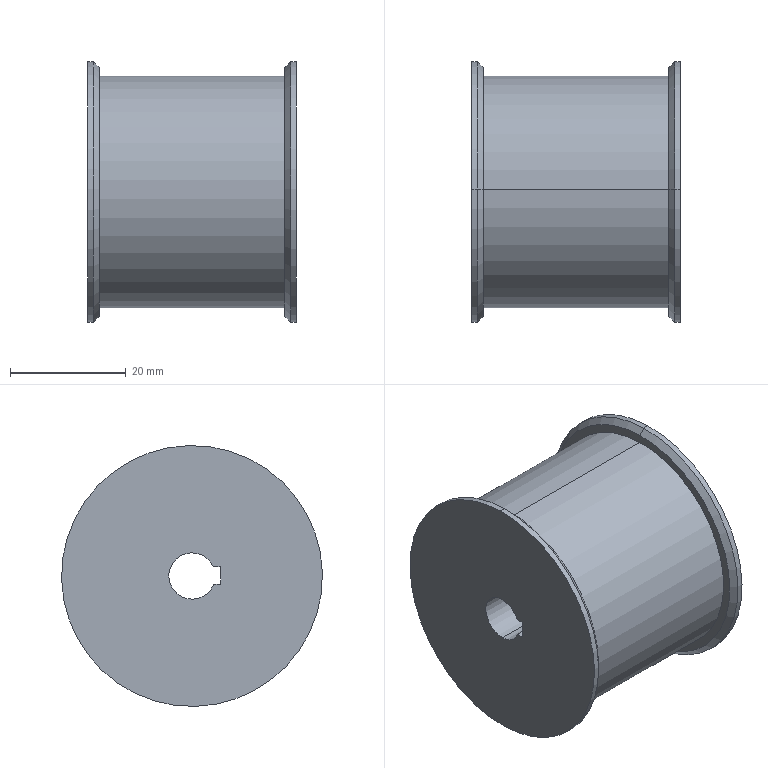Component | SolidWorks | CHEN123-AA-13-1 | 1 solid | 20 faces | box 36 x 45 x 45 mm | volume 44517 mm3 | cylinder 9 | plane 7 | cone 4 | commonest cylinder face diameters 45 x4 8 x3 40 x2
build123d program:
from build123d import *

# Parameters (mm, degrees)
SKETCH1_R           = 20
BOSS_EXTRUDE1_DEPTH = 16
SKETCH2_R           = 22.5
BOSS_EXTRUDE2_DEPTH = 2
BOSS_EXTRUDE3_START = 2
SKETCH3_R           = 22.5
BOSS_EXTRUDE3_DEPTH = 2
CHAMFER1_SIZE       = 1
SKETCH4_R           = 4
CUT_EXTRUDE1_DEPTH  = 49.047
SKETCH5_W           = 3
SKETCH5_H           = 1.816
CUT_EXTRUDE2_DEPTH  = 49.047


with BuildPart() as part:
    # Sketch1 → Boss-Extrude1 (new, symmetric)
    with BuildSketch(Plane.XY):
        Circle(SKETCH1_R)
    extrude(amount=BOSS_EXTRUDE1_DEPTH, both=True)

    # Sketch2 → Boss-Extrude2 (add)
    with BuildSketch(Plane.XY.offset(16)):
        Circle(SKETCH2_R)
    extrude(amount=BOSS_EXTRUDE2_DEPTH)

    # Sketch3 → Boss-Extrude3 (add)
    with BuildSketch(Plane(origin=(0, 0, -16), x_dir=(-1, 0, 0), z_dir=(0, 0, -1)).offset(BOSS_EXTRUDE3_START)):
        with Locations(Location((0, 0, 0), (0, 0, 180))):
            Circle(SKETCH3_R)
    extrude(amount=-BOSS_EXTRUDE3_DEPTH)

    # Chamfer1
    chamfer1_edges = [part.edges().sort_by_distance(p)[0] for p in [
        (-22.5, 0, 16),
        (-22.5, 0, -16),
    ]]
    chamfer(chamfer1_edges, length=CHAMFER1_SIZE)

    # Sketch4 → Cut-Extrude1 (cut, through all)
    with BuildSketch(Plane(origin=(0, 0, -18), x_dir=(-1, 0, 0), z_dir=(0, 0, -1))):
        Circle(SKETCH4_R)
    extrude(amount=-CUT_EXTRUDE1_DEPTH, mode=Mode.SUBTRACT)

    # Sketch5 → Cut-Extrude2 (cut, through all)
    with BuildSketch(Plane(origin=(0, 0, -18), x_dir=(-1, 0, 0), z_dir=(0, 0, -1))):
        with Locations((0, 4)):
            Rectangle(SKETCH5_W, SKETCH5_H)
    extrude(amount=-CUT_EXTRUDE2_DEPTH, mode=Mode.SUBTRACT)


solid = part.part

# Placed as in the assembly
solid = solid.moved(Location((-0.0005, -95.999, -200), (178.787, -90, 0)))
STEP:
#1=CARTESIAN_POINT('',(-0.7087,-3.783,-8.031));
#2=VERTEX_POINT('',#1);
#3=CARTESIAN_POINT('',(-0.7087,-3.776,-7.717));
#4=VERTEX_POINT('',#3);
#5=CARTESIAN_POINT('',(-0.7087,-3.779,-7.874));
#6=DIRECTION('',(1.,0.,0.));
#7=DIRECTION('',(0.,0.02117,0.9998));
#8=AXIS2_PLACEMENT_3D('',#5,#6,#7);
#9=CIRCLE('',#8,0.1575);
#10=EDGE_CURVE('',#2,#4,#9,.T.);
#11=ORIENTED_EDGE('',*,*,#10,.F.);
#12=CARTESIAN_POINT('',(0.7086,-3.783,-8.031));
#13=VERTEX_POINT('',#12);
#14=CARTESIAN_POINT('',(-0.7087,-3.783,-8.031));
#15=DIRECTION('',(1.,0.,0.));
#16=VECTOR('',#15,39.37);
#17=LINE('',#14,#16);
#18=EDGE_CURVE('',#2,#13,#17,.T.);
#19=ORIENTED_EDGE('',*,*,#18,.T.);
#20=CARTESIAN_POINT('',(0.7086,-3.776,-7.717));
#21=VERTEX_POINT('',#20);
#22=CARTESIAN_POINT('',(0.7086,-3.779,-7.874));
#23=DIRECTION('',(1.,0.,0.));
#24=DIRECTION('',(0.,0.02117,0.9998));
#25=AXIS2_PLACEMENT_3D('',#22,#23,#24);
#26=CIRCLE('',#25,0.1575);
#27=EDGE_CURVE('',#13,#21,#26,.T.);
#28=ORIENTED_EDGE('',*,*,#27,.T.);
#29=CARTESIAN_POINT('',(-0.7087,-3.776,-7.717));
#30=DIRECTION('',(1.,0.,0.));
#31=VECTOR('',#30,39.37);
#32=LINE('',#29,#31);
#33=EDGE_CURVE('',#4,#21,#32,.T.);
#34=ORIENTED_EDGE('',*,*,#33,.F.);
#35=EDGE_LOOP('',(#11,#19,#28,#34));
#36=FACE_OUTER_BOUND('',#35,.T.);
#37=CARTESIAN_POINT('',(-0.7087,-3.779,-7.874));
#38=DIRECTION('',(1.,0.,0.));
#39=DIRECTION('',(0.,0.02117,0.9998));
#40=AXIS2_PLACEMENT_3D('',#37,#38,#39);
#41=CYLINDRICAL_SURFACE('',#40,0.1575);
#42=ADVANCED_FACE('',(#36),#41,.F.);
#43=CARTESIAN_POINT('',(-0.7087,-3.924,-7.812));
#44=VERTEX_POINT('',#43);
#45=CARTESIAN_POINT('',(-0.7087,-3.779,-7.874));
#46=DIRECTION('',(1.,0.,0.));
#47=DIRECTION('',(0.,0.02117,0.9998));
#48=AXIS2_PLACEMENT_3D('',#45,#46,#47);
#49=CIRCLE('',#48,0.1575);
#50=EDGE_CURVE('',#4,#44,#49,.T.);
#51=ORIENTED_EDGE('',*,*,#50,.F.);
#52=ORIENTED_EDGE('',*,*,#33,.T.);
#53=CARTESIAN_POINT('',(0.7086,-3.924,-7.812));
#54=VERTEX_POINT('',#53);
#55=CARTESIAN_POINT('',(0.7086,-3.779,-7.874));
#56=DIRECTION('',(1.,0.,0.));
#57=DIRECTION('',(0.,0.02117,0.9998));
#58=AXIS2_PLACEMENT_3D('',#55,#56,#57);
#59=CIRCLE('',#58,0.1575);
#60=EDGE_CURVE('',#21,#54,#59,.T.);
#61=ORIENTED_EDGE('',*,*,#60,.T.);
#62=CARTESIAN_POINT('',(-0.7087,-3.924,-7.812));
#63=DIRECTION('',(-1.,0.,0.));
#64=VECTOR('',#63,39.37);
#65=LINE('',#62,#64);
#66=EDGE_CURVE('',#54,#44,#65,.T.);
#67=ORIENTED_EDGE('',*,*,#66,.T.);
#68=EDGE_LOOP('',(#51,#52,#61,#67));
#69=FACE_OUTER_BOUND('',#68,.T.);
#70=CARTESIAN_POINT('',(-0.7087,-3.779,-7.874));
#71=DIRECTION('',(1.,0.,0.));
#72=DIRECTION('',(0.,0.02117,0.9998));
#73=AXIS2_PLACEMENT_3D('',#70,#71,#72);
#74=CYLINDRICAL_SURFACE('',#73,0.1575);
#75=ADVANCED_FACE('',(#69),#74,.F.);
#76=CARTESIAN_POINT('',(-0.6299,-3.762,-7.028));
#77=VERTEX_POINT('',#76);
#78=CARTESIAN_POINT('',(-0.6299,-3.797,-8.72));
#79=VERTEX_POINT('',#78);
#80=CARTESIAN_POINT('',(-0.6299,-3.779,-7.874));
#81=DIRECTION('',(1.,0.,0.));
#82=DIRECTION('',(0.,-0.02117,-0.9998));
#83=AXIS2_PLACEMENT_3D('',#80,#81,#82);
#84=CIRCLE('',#83,0.8465);
#85=EDGE_CURVE('',#77,#79,#84,.T.);
#86=ORIENTED_EDGE('',*,*,#85,.F.);
#87=CARTESIAN_POINT('',(-0.6693,-3.761,-6.988));
#88=VERTEX_POINT('',#87);
#89=CARTESIAN_POINT('',(-0.6693,-3.761,-6.988));
#90=DIRECTION('',(-0.7071,0.01497,0.7069));
#91=VECTOR('',#90,39.37);
#92=LINE('',#89,#91);
#93=EDGE_CURVE('',#77,#88,#92,.T.);
#94=ORIENTED_EDGE('',*,*,#93,.T.);
#95=CARTESIAN_POINT('',(-0.6693,-3.798,-8.76));
#96=VERTEX_POINT('',#95);
#97=CARTESIAN_POINT('',(-0.6693,-3.779,-7.874));
#98=DIRECTION('',(-1.,0.,0.));
#99=DIRECTION('',(0.,-0.02117,-0.9998));
#100=AXIS2_PLACEMENT_3D('',#97,#98,#99);
#101=CIRCLE('',#100,0.8858);
#102=EDGE_CURVE('',#96,#88,#101,.T.);
#103=ORIENTED_EDGE('',*,*,#102,.F.);
#104=CARTESIAN_POINT('',(-0.6693,-3.798,-8.76));
#105=DIRECTION('',(-0.7071,-0.01497,-0.7069));
#106=VECTOR('',#105,39.37);
#107=LINE('',#104,#106);
#108=EDGE_CURVE('',#79,#96,#107,.T.);
#109=ORIENTED_EDGE('',*,*,#108,.F.);
#110=EDGE_LOOP('',(#86,#94,#103,#109));
#111=FACE_OUTER_BOUND('',#110,.T.);
#112=CARTESIAN_POINT('',(-0.6693,-3.779,-7.874));
#113=DIRECTION('',(-1.,0.,0.));
#114=DIRECTION('',(0.,-0.02117,-0.9998));
#115=AXIS2_PLACEMENT_3D('',#112,#113,#114);
#116=CONICAL_SURFACE('',#115,0.8858,0.7854);
#117=ADVANCED_FACE('',(#111),#116,.T.);
#118=CARTESIAN_POINT('',(0.6299,-3.797,-8.72));
#119=VERTEX_POINT('',#118);
#120=CARTESIAN_POINT('',(0.6299,-3.762,-7.028));
#121=VERTEX_POINT('',#120);
#122=CARTESIAN_POINT('',(0.6299,-3.779,-7.874));
#123=DIRECTION('',(-1.,0.,0.));
#124=DIRECTION('',(0.,0.02117,0.9998));
#125=AXIS2_PLACEMENT_3D('',#122,#123,#124);
#126=CIRCLE('',#125,0.8465);
#127=EDGE_CURVE('',#119,#121,#126,.T.);
#128=ORIENTED_EDGE('',*,*,#127,.F.);
#129=CARTESIAN_POINT('',(0.6693,-3.798,-8.76));
#130=VERTEX_POINT('',#129);
#131=CARTESIAN_POINT('',(0.6693,-3.798,-8.76));
#132=DIRECTION('',(0.7071,-0.01497,-0.7069));
#133=VECTOR('',#132,39.37);
#134=LINE('',#131,#133);
#135=EDGE_CURVE('',#119,#130,#134,.T.);
#136=ORIENTED_EDGE('',*,*,#135,.T.);
#137=CARTESIAN_POINT('',(0.6693,-3.761,-6.988));
#138=VERTEX_POINT('',#137);
#139=CARTESIAN_POINT('',(0.6693,-3.779,-7.874));
#140=DIRECTION('',(1.,0.,0.));
#141=DIRECTION('',(0.,0.02117,0.9998));
#142=AXIS2_PLACEMENT_3D('',#139,#140,#141);
#143=CIRCLE('',#142,0.8858);
#144=EDGE_CURVE('',#138,#130,#143,.T.);
#145=ORIENTED_EDGE('',*,*,#144,.F.);
#146=CARTESIAN_POINT('',(0.6693,-3.761,-6.988));
#147=DIRECTION('',(0.7071,0.01497,0.7069));
#148=VECTOR('',#147,39.37);
#149=LINE('',#146,#148);
#150=EDGE_CURVE('',#121,#138,#149,.T.);
#151=ORIENTED_EDGE('',*,*,#150,.F.);
#152=EDGE_LOOP('',(#128,#136,#145,#151));
#153=FACE_OUTER_BOUND('',#152,.T.);
#154=CARTESIAN_POINT('',(0.6693,-3.779,-7.874));
#155=DIRECTION('',(1.,0.,0.));
#156=DIRECTION('',(0.,0.02117,0.9998));
#157=AXIS2_PLACEMENT_3D('',#154,#155,#156);
#158=CONICAL_SURFACE('',#157,0.8858,0.7854);
#159=ADVANCED_FACE('',(#153),#158,.T.);
#160=CARTESIAN_POINT('',(0.7086,-3.761,-6.988));
#161=VERTEX_POINT('',#160);
#162=CARTESIAN_POINT('',(0.7086,-3.798,-8.76));
#163=VERTEX_POINT('',#162);
#164=CARTESIAN_POINT('',(0.7086,-3.779,-7.874));
#165=DIRECTION('',(1.,0.,0.));
#166=DIRECTION('',(0.,0.02117,0.9998));
#167=AXIS2_PLACEMENT_3D('',#164,#165,#166);
#168=CIRCLE('',#167,0.8858);
#169=EDGE_CURVE('',#161,#163,#168,.T.);
#170=ORIENTED_EDGE('',*,*,#169,.F.);
#171=CARTESIAN_POINT('',(0.7086,-3.761,-6.988));
#172=DIRECTION('',(-1.,0.,0.));
#173=VECTOR('',#172,39.37);
#174=LINE('',#171,#173);
#175=EDGE_CURVE('',#161,#138,#174,.T.);
#176=ORIENTED_EDGE('',*,*,#175,.T.);
#177=ORIENTED_EDGE('',*,*,#144,.T.);
#178=CARTESIAN_POINT('',(0.7086,-3.798,-8.76));
#179=DIRECTION('',(-1.,0.,0.));
#180=VECTOR('',#179,39.37);
#181=LINE('',#178,#180);
#182=EDGE_CURVE('',#163,#130,#181,.T.);
#183=ORIENTED_EDGE('',*,*,#182,.F.);
#184=EDGE_LOOP('',(#170,#176,#177,#183));
#185=FACE_OUTER_BOUND('',#184,.T.);
#186=CARTESIAN_POINT('',(0.7086,-3.779,-7.874));
#187=DIRECTION('',(-1.,0.,0.));
#188=DIRECTION('',(0.,-0.02117,-0.9998));
#189=AXIS2_PLACEMENT_3D('',#186,#187,#188);
#190=CYLINDRICAL_SURFACE('',#189,0.8858);
#191=ADVANCED_FACE('',(#185),#190,.T.);
#192=CARTESIAN_POINT('',(-0.7087,-3.798,-8.76));
#193=VERTEX_POINT('',#192);
#194=CARTESIAN_POINT('',(-0.7087,-3.761,-6.988));
#195=VERTEX_POINT('',#194);
#196=CARTESIAN_POINT('',(-0.7087,-3.779,-7.874));
#197=DIRECTION('',(-1.,0.,0.));
#198=DIRECTION('',(0.,-0.02117,-0.9998));
#199=AXIS2_PLACEMENT_3D('',#196,#197,#198);
#200=CIRCLE('',#199,0.8858);
#201=EDGE_CURVE('',#193,#195,#200,.T.);
#202=ORIENTED_EDGE('',*,*,#201,.F.);
#203=CARTESIAN_POINT('',(-0.7087,-3.798,-8.76));
#204=DIRECTION('',(1.,0.,0.));
#205=VECTOR('',#204,39.37);
#206=LINE('',#203,#205);
#207=EDGE_CURVE('',#193,#96,#206,.T.);
#208=ORIENTED_EDGE('',*,*,#207,.T.);
#209=ORIENTED_EDGE('',*,*,#102,.T.);
#210=CARTESIAN_POINT('',(-0.7087,-3.761,-6.988));
#211=DIRECTION('',(1.,0.,0.));
#212=VECTOR('',#211,39.37);
#213=LINE('',#210,#212);
#214=EDGE_CURVE('',#195,#88,#213,.T.);
#215=ORIENTED_EDGE('',*,*,#214,.F.);
#216=EDGE_LOOP('',(#202,#208,#209,#215));
#217=FACE_OUTER_BOUND('',#216,.T.);
#218=CARTESIAN_POINT('',(-0.7087,-3.779,-7.874));
#219=DIRECTION('',(1.,0.,0.));
#220=DIRECTION('',(0.,0.02117,0.9998));
#221=AXIS2_PLACEMENT_3D('',#218,#219,#220);
#222=CYLINDRICAL_SURFACE('',#221,0.8858);
#223=ADVANCED_FACE('',(#217),#222,.T.);
#224=CARTESIAN_POINT('',(-0.6299,-3.796,-8.661));
#225=VERTEX_POINT('',#224);
#226=CARTESIAN_POINT('',(-0.6299,-3.763,-7.087));
#227=VERTEX_POINT('',#226);
#228=CARTESIAN_POINT('',(-0.6299,-3.779,-7.874));
#229=DIRECTION('',(-1.,0.,0.));
#230=DIRECTION('',(0.,-0.02117,-0.9998));
#231=AXIS2_PLACEMENT_3D('',#228,#229,#230);
#232=CIRCLE('',#231,0.7874);
#233=EDGE_CURVE('',#225,#227,#232,.T.);
#234=ORIENTED_EDGE('',*,*,#233,.F.);
#235=CARTESIAN_POINT('',(0.6299,-3.796,-8.661));
#236=VERTEX_POINT('',#235);
#237=CARTESIAN_POINT('',(-0.6299,-3.796,-8.661));
#238=DIRECTION('',(1.,0.,0.));
#239=VECTOR('',#238,39.37);
#240=LINE('',#237,#239);
#241=EDGE_CURVE('',#225,#236,#240,.T.);
#242=ORIENTED_EDGE('',*,*,#241,.T.);
#243=CARTESIAN_POINT('',(0.6299,-3.763,-7.087));
#244=VERTEX_POINT('',#243);
#245=CARTESIAN_POINT('',(0.6299,-3.779,-7.874));
#246=DIRECTION('',(-1.,0.,0.));
#247=DIRECTION('',(0.,-0.02117,-0.9998));
#248=AXIS2_PLACEMENT_3D('',#245,#246,#247);
#249=CIRCLE('',#248,0.7874);
#250=EDGE_CURVE('',#236,#244,#249,.T.);
#251=ORIENTED_EDGE('',*,*,#250,.T.);
#252=CARTESIAN_POINT('',(-0.6299,-3.763,-7.087));
#253=DIRECTION('',(1.,0.,0.));
#254=VECTOR('',#253,39.37);
#255=LINE('',#252,#254);
#256=EDGE_CURVE('',#227,#244,#255,.T.);
#257=ORIENTED_EDGE('',*,*,#256,.F.);
#258=EDGE_LOOP('',(#234,#242,#251,#257));
#259=FACE_OUTER_BOUND('',#258,.T.);
#260=CARTESIAN_POINT('',(-0.6299,-3.779,-7.874));
#261=DIRECTION('',(1.,0.,0.));
#262=DIRECTION('',(0.,0.02117,0.9998));
#263=AXIS2_PLACEMENT_3D('',#260,#261,#262);
#264=CYLINDRICAL_SURFACE('',#263,0.7874);
#265=ADVANCED_FACE('',(#259),#264,.T.);
#266=ORIENTED_EDGE('',*,*,#241,.F.);
#267=CARTESIAN_POINT('',(-0.6299,-3.779,-7.874));
#268=DIRECTION('',(-1.,0.,0.));
#269=DIRECTION('',(0.,-0.02117,-0.9998));
#270=AXIS2_PLACEMENT_3D('',#267,#268,#269);
#271=CIRCLE('',#270,0.7874);
#272=EDGE_CURVE('',#227,#225,#271,.T.);
#273=ORIENTED_EDGE('',*,*,#272,.F.);
#274=ORIENTED_EDGE('',*,*,#256,.T.);
#275=CARTESIAN_POINT('',(0.6299,-3.779,-7.874));
#276=DIRECTION('',(-1.,0.,0.));
#277=DIRECTION('',(0.,-0.02117,-0.9998));
#278=AXIS2_PLACEMENT_3D('',#275,#276,#277);
#279=CIRCLE('',#278,0.7874);
#280=EDGE_CURVE('',#244,#236,#279,.T.);
#281=ORIENTED_EDGE('',*,*,#280,.T.);
#282=EDGE_LOOP('',(#266,#273,#274,#281));
#283=FACE_OUTER_BOUND('',#282,.T.);
#284=CARTESIAN_POINT('',(-0.6299,-3.779,-7.874));
#285=DIRECTION('',(1.,0.,0.));
#286=DIRECTION('',(0.,0.02117,0.9998));
#287=AXIS2_PLACEMENT_3D('',#284,#285,#286);
#288=CYLINDRICAL_SURFACE('',#287,0.7874);
#289=ADVANCED_FACE('',(#283),#288,.T.);
#290=ORIENTED_EDGE('',*,*,#207,.F.);
#291=CARTESIAN_POINT('',(-0.7087,-3.779,-7.874));
#292=DIRECTION('',(-1.,0.,0.));
#293=DIRECTION('',(0.,-0.02117,-0.9998));
#294=AXIS2_PLACEMENT_3D('',#291,#292,#293);
#295=CIRCLE('',#294,0.8858);
#296=EDGE_CURVE('',#195,#193,#295,.T.);
#297=ORIENTED_EDGE('',*,*,#296,.F.);
#298=ORIENTED_EDGE('',*,*,#214,.T.);
#299=CARTESIAN_POINT('',(-0.6693,-3.779,-7.874));
#300=DIRECTION('',(-1.,0.,0.));
#301=DIRECTION('',(0.,-0.02117,-0.9998));
#302=AXIS2_PLACEMENT_3D('',#299,#300,#301);
#303=CIRCLE('',#302,0.8858);
#304=EDGE_CURVE('',#88,#96,#303,.T.);
#305=ORIENTED_EDGE('',*,*,#304,.T.);
#306=EDGE_LOOP('',(#290,#297,#298,#305));
#307=FACE_OUTER_BOUND('',#306,.T.);
#308=CARTESIAN_POINT('',(-0.7087,-3.779,-7.874));
#309=DIRECTION('',(1.,0.,0.));
#310=DIRECTION('',(0.,0.02117,0.9998));
#311=AXIS2_PLACEMENT_3D('',#308,#309,#310);
#312=CYLINDRICAL_SURFACE('',#311,0.8858);
#313=ADVANCED_FACE('',(#307),#312,.T.);
#314=CARTESIAN_POINT('',(-0.7087,-3.971,-7.811));
#315=VERTEX_POINT('',#314);
#316=CARTESIAN_POINT('',(-0.7087,-3.9,-7.812));
#317=DIRECTION('',(0.,-0.9998,0.02117));
#318=VECTOR('',#317,39.37);
#319=LINE('',#316,#318);
#320=EDGE_CURVE('',#44,#315,#319,.T.);
#321=ORIENTED_EDGE('',*,*,#320,.T.);
#322=CARTESIAN_POINT('',(-0.7087,-3.974,-7.929));
#323=VERTEX_POINT('',#322);
#324=CARTESIAN_POINT('',(-0.7087,-3.974,-7.929));
#325=DIRECTION('',(0.,-0.02117,-0.9998));
#326=VECTOR('',#325,39.37);
#327=LINE('',#324,#326);
#328=EDGE_CURVE('',#315,#323,#327,.T.);
#329=ORIENTED_EDGE('',*,*,#328,.T.);
#330=CARTESIAN_POINT('',(-0.7087,-3.927,-7.93));
#331=VERTEX_POINT('',#330);
#332=CARTESIAN_POINT('',(-0.7087,-3.902,-7.93));
#333=DIRECTION('',(0.,0.9998,-0.02117));
#334=VECTOR('',#333,39.37);
#335=LINE('',#332,#334);
#336=EDGE_CURVE('',#323,#331,#335,.T.);
#337=ORIENTED_EDGE('',*,*,#336,.T.);
#338=CARTESIAN_POINT('',(-0.7087,-3.779,-7.874));
#339=DIRECTION('',(1.,0.,0.));
#340=DIRECTION('',(0.,0.02117,0.9998));
#341=AXIS2_PLACEMENT_3D('',#338,#339,#340);
#342=CIRCLE('',#341,0.1575);
#343=EDGE_CURVE('',#331,#2,#342,.T.);
#344=ORIENTED_EDGE('',*,*,#343,.T.);
#345=ORIENTED_EDGE('',*,*,#10,.T.);
#346=ORIENTED_EDGE('',*,*,#50,.T.);
#347=EDGE_LOOP('',(#321,#329,#337,#344,#345,#346));
#348=FACE_BOUND('',#347,.T.);
#349=ORIENTED_EDGE('',*,*,#296,.T.);
#350=ORIENTED_EDGE('',*,*,#201,.T.);
#351=EDGE_LOOP('',(#349,#350));
#352=FACE_OUTER_BOUND('',#351,.T.);
#353=CARTESIAN_POINT('',(-0.7087,-3.779,-7.874));
#354=DIRECTION('',(-1.,0.,0.));
#355=DIRECTION('',(0.,-0.02117,-0.9998));
#356=AXIS2_PLACEMENT_3D('',#353,#354,#355);
#357=PLANE('',#356);
#358=ADVANCED_FACE('',(#348,#352),#357,.T.);
#359=CARTESIAN_POINT('',(-0.6299,-3.779,-7.874));
#360=DIRECTION('',(1.,0.,0.));
#361=DIRECTION('',(0.,-0.02117,-0.9998));
#362=AXIS2_PLACEMENT_3D('',#359,#360,#361);
#363=CIRCLE('',#362,0.8465);
#364=EDGE_CURVE('',#79,#77,#363,.T.);
#365=ORIENTED_EDGE('',*,*,#364,.T.);
#366=ORIENTED_EDGE('',*,*,#85,.T.);
#367=EDGE_LOOP('',(#365,#366));
#368=FACE_OUTER_BOUND('',#367,.T.);
#369=ORIENTED_EDGE('',*,*,#272,.T.);
#370=ORIENTED_EDGE('',*,*,#233,.T.);
#371=EDGE_LOOP('',(#369,#370));
#372=FACE_BOUND('',#371,.T.);
#373=CARTESIAN_POINT('',(-0.6299,-3.779,-7.874));
#374=DIRECTION('',(-1.,0.,0.));
#375=DIRECTION('',(0.,-0.02117,-0.9998));
#376=AXIS2_PLACEMENT_3D('',#373,#374,#375);
#377=PLANE('',#376);
#378=ADVANCED_FACE('',(#368,#372),#377,.F.);
#379=ORIENTED_EDGE('',*,*,#175,.F.);
#380=CARTESIAN_POINT('',(0.7086,-3.779,-7.874));
#381=DIRECTION('',(1.,0.,0.));
#382=DIRECTION('',(0.,0.02117,0.9998));
#383=AXIS2_PLACEMENT_3D('',#380,#381,#382);
#384=CIRCLE('',#383,0.8858);
#385=EDGE_CURVE('',#163,#161,#384,.T.);
#386=ORIENTED_EDGE('',*,*,#385,.F.);
#387=ORIENTED_EDGE('',*,*,#182,.T.);
#388=CARTESIAN_POINT('',(0.6693,-3.779,-7.874));
#389=DIRECTION('',(1.,0.,0.));
#390=DIRECTION('',(0.,0.02117,0.9998));
#391=AXIS2_PLACEMENT_3D('',#388,#389,#390);
#392=CIRCLE('',#391,0.8858);
#393=EDGE_CURVE('',#130,#138,#392,.T.);
#394=ORIENTED_EDGE('',*,*,#393,.T.);
#395=EDGE_LOOP('',(#379,#386,#387,#394));
#396=FACE_OUTER_BOUND('',#395,.T.);
#397=CARTESIAN_POINT('',(0.7086,-3.779,-7.874));
#398=DIRECTION('',(-1.,0.,0.));
#399=DIRECTION('',(0.,-0.02117,-0.9998));
#400=AXIS2_PLACEMENT_3D('',#397,#398,#399);
#401=CYLINDRICAL_SURFACE('',#400,0.8858);
#402=ADVANCED_FACE('',(#396),#401,.T.);
#403=CARTESIAN_POINT('',(0.7086,-3.971,-7.811));
#404=VERTEX_POINT('',#403);
#405=CARTESIAN_POINT('',(0.7086,-3.9,-7.812));
#406=DIRECTION('',(0.,-0.9998,0.02117));
#407=VECTOR('',#406,39.37);
#408=LINE('',#405,#407);
#409=EDGE_CURVE('',#54,#404,#408,.T.);
#410=ORIENTED_EDGE('',*,*,#409,.F.);
#411=ORIENTED_EDGE('',*,*,#60,.F.);
#412=ORIENTED_EDGE('',*,*,#27,.F.);
#413=CARTESIAN_POINT('',(0.7086,-3.927,-7.93));
#414=VERTEX_POINT('',#413);
#415=CARTESIAN_POINT('',(0.7086,-3.779,-7.874));
#416=DIRECTION('',(1.,0.,0.));
#417=DIRECTION('',(0.,0.02117,0.9998));
#418=AXIS2_PLACEMENT_3D('',#415,#416,#417);
#419=CIRCLE('',#418,0.1575);
#420=EDGE_CURVE('',#414,#13,#419,.T.);
#421=ORIENTED_EDGE('',*,*,#420,.F.);
#422=CARTESIAN_POINT('',(0.7086,-3.974,-7.929));
#423=VERTEX_POINT('',#422);
#424=CARTESIAN_POINT('',(0.7086,-3.902,-7.93));
#425=DIRECTION('',(0.,0.9998,-0.02117));
#426=VECTOR('',#425,39.37);
#427=LINE('',#424,#426);
#428=EDGE_CURVE('',#423,#414,#427,.T.);
#429=ORIENTED_EDGE('',*,*,#428,.F.);
#430=CARTESIAN_POINT('',(0.7086,-3.974,-7.929));
#431=DIRECTION('',(0.,-0.02117,-0.9998));
#432=VECTOR('',#431,39.37);
#433=LINE('',#430,#432);
#434=EDGE_CURVE('',#404,#423,#433,.T.);
#435=ORIENTED_EDGE('',*,*,#434,.F.);
#436=EDGE_LOOP('',(#410,#411,#412,#421,#429,#435));
#437=FACE_BOUND('',#436,.T.);
#438=ORIENTED_EDGE('',*,*,#385,.T.);
#439=ORIENTED_EDGE('',*,*,#169,.T.);
#440=EDGE_LOOP('',(#438,#439));
#441=FACE_OUTER_BOUND('',#440,.T.);
#442=CARTESIAN_POINT('',(0.7086,-3.779,-7.874));
#443=DIRECTION('',(1.,0.,0.));
#444=DIRECTION('',(0.,0.02117,0.9998));
#445=AXIS2_PLACEMENT_3D('',#442,#443,#444);
#446=PLANE('',#445);
#447=ADVANCED_FACE('',(#437,#441),#446,.T.);
#448=CARTESIAN_POINT('',(0.6299,-3.779,-7.874));
#449=DIRECTION('',(-1.,0.,0.));
#450=DIRECTION('',(0.,0.02117,0.9998));
#451=AXIS2_PLACEMENT_3D('',#448,#449,#450);
#452=CIRCLE('',#451,0.8465);
#453=EDGE_CURVE('',#121,#119,#452,.T.);
#454=ORIENTED_EDGE('',*,*,#453,.T.);
#455=ORIENTED_EDGE('',*,*,#127,.T.);
#456=EDGE_LOOP('',(#454,#455));
#457=FACE_OUTER_BOUND('',#456,.T.);
#458=ORIENTED_EDGE('',*,*,#280,.F.);
#459=ORIENTED_EDGE('',*,*,#250,.F.);
#460=EDGE_LOOP('',(#458,#459));
#461=FACE_BOUND('',#460,.T.);
#462=CARTESIAN_POINT('',(0.6299,-3.779,-7.874));
#463=DIRECTION('',(1.,0.,0.));
#464=DIRECTION('',(0.,0.02117,0.9998));
#465=AXIS2_PLACEMENT_3D('',#462,#463,#464);
#466=PLANE('',#465);
#467=ADVANCED_FACE('',(#457,#461),#466,.F.);
#468=ORIENTED_EDGE('',*,*,#135,.F.);
#469=ORIENTED_EDGE('',*,*,#453,.F.);
#470=ORIENTED_EDGE('',*,*,#150,.T.);
#471=ORIENTED_EDGE('',*,*,#393,.F.);
#472=EDGE_LOOP('',(#468,#469,#470,#471));
#473=FACE_OUTER_BOUND('',#472,.T.);
#474=CARTESIAN_POINT('',(0.6693,-3.779,-7.874));
#475=DIRECTION('',(1.,0.,0.));
#476=DIRECTION('',(0.,0.02117,0.9998));
#477=AXIS2_PLACEMENT_3D('',#474,#475,#476);
#478=CONICAL_SURFACE('',#477,0.8858,0.7854);
#479=ADVANCED_FACE('',(#473),#478,.T.);
#480=ORIENTED_EDGE('',*,*,#93,.F.);
#481=ORIENTED_EDGE('',*,*,#364,.F.);
#482=ORIENTED_EDGE('',*,*,#108,.T.);
#483=ORIENTED_EDGE('',*,*,#304,.F.);
#484=EDGE_LOOP('',(#480,#481,#482,#483));
#485=FACE_OUTER_BOUND('',#484,.T.);
#486=CARTESIAN_POINT('',(-0.6693,-3.779,-7.874));
#487=DIRECTION('',(-1.,0.,0.));
#488=DIRECTION('',(0.,-0.02117,-0.9998));
#489=AXIS2_PLACEMENT_3D('',#486,#487,#488);
#490=CONICAL_SURFACE('',#489,0.8858,0.7854);
#491=ADVANCED_FACE('',(#485),#490,.T.);
#492=ORIENTED_EDGE('',*,*,#18,.F.);
#493=ORIENTED_EDGE('',*,*,#343,.F.);
#494=CARTESIAN_POINT('',(-0.7087,-3.927,-7.93));
#495=DIRECTION('',(1.,0.,0.));
#496=VECTOR('',#495,39.37);
#497=LINE('',#494,#496);
#498=EDGE_CURVE('',#331,#414,#497,.T.);
#499=ORIENTED_EDGE('',*,*,#498,.T.);
#500=ORIENTED_EDGE('',*,*,#420,.T.);
#501=EDGE_LOOP('',(#492,#493,#499,#500));
#502=FACE_OUTER_BOUND('',#501,.T.);
#503=CARTESIAN_POINT('',(-0.7087,-3.779,-7.874));
#504=DIRECTION('',(1.,0.,0.));
#505=DIRECTION('',(0.,0.02117,0.9998));
#506=AXIS2_PLACEMENT_3D('',#503,#504,#505);
#507=CYLINDRICAL_SURFACE('',#506,0.1575);
#508=ADVANCED_FACE('',(#502),#507,.F.);
#509=ORIENTED_EDGE('',*,*,#409,.T.);
#510=CARTESIAN_POINT('',(-0.7087,-3.971,-7.811));
#511=DIRECTION('',(1.,0.,0.));
#512=VECTOR('',#511,39.37);
#513=LINE('',#510,#512);
#514=EDGE_CURVE('',#315,#404,#513,.T.);
#515=ORIENTED_EDGE('',*,*,#514,.F.);
#516=ORIENTED_EDGE('',*,*,#320,.F.);
#517=ORIENTED_EDGE('',*,*,#66,.F.);
#518=EDGE_LOOP('',(#509,#515,#516,#517));
#519=FACE_OUTER_BOUND('',#518,.T.);
#520=CARTESIAN_POINT('',(-0.7087,-3.9,-7.812));
#521=DIRECTION('',(0.,0.02117,0.9998));
#522=DIRECTION('',(-1.,0.,0.));
#523=AXIS2_PLACEMENT_3D('',#520,#521,#522);
#524=PLANE('',#523);
#525=ADVANCED_FACE('',(#519),#524,.F.);
#526=ORIENTED_EDGE('',*,*,#336,.F.);
#527=CARTESIAN_POINT('',(-0.7087,-3.974,-7.929));
#528=DIRECTION('',(1.,0.,0.));
#529=VECTOR('',#528,39.37);
#530=LINE('',#527,#529);
#531=EDGE_CURVE('',#323,#423,#530,.T.);
#532=ORIENTED_EDGE('',*,*,#531,.T.);
#533=ORIENTED_EDGE('',*,*,#428,.T.);
#534=ORIENTED_EDGE('',*,*,#498,.F.);
#535=EDGE_LOOP('',(#526,#532,#533,#534));
#536=FACE_OUTER_BOUND('',#535,.T.);
#537=CARTESIAN_POINT('',(-0.7087,-3.902,-7.93));
#538=DIRECTION('',(0.,-0.02117,-0.9998));
#539=DIRECTION('',(1.,0.,0.));
#540=AXIS2_PLACEMENT_3D('',#537,#538,#539);
#541=PLANE('',#540);
#542=ADVANCED_FACE('',(#536),#541,.F.);
#543=ORIENTED_EDGE('',*,*,#434,.T.);
#544=ORIENTED_EDGE('',*,*,#531,.F.);
#545=ORIENTED_EDGE('',*,*,#328,.F.);
#546=ORIENTED_EDGE('',*,*,#514,.T.);
#547=EDGE_LOOP('',(#543,#544,#545,#546));
#548=FACE_OUTER_BOUND('',#547,.T.);
#549=CARTESIAN_POINT('',(-0.7087,-3.974,-7.929));
#550=DIRECTION('',(0.,-0.9998,0.02117));
#551=DIRECTION('',(-1.,0.,0.));
#552=AXIS2_PLACEMENT_3D('',#549,#550,#551);
#553=PLANE('',#552);
#554=ADVANCED_FACE('',(#548),#553,.F.);
#555=CLOSED_SHELL('',(#42,#75,#117,#159,#191,#223,#265,#289,#313,#358,#378,#402,#447,#467,#479,#491,#508,#525,#542,#554));
#556=MANIFOLD_SOLID_BREP('',#555);
#557=CARTESIAN_POINT('',(0.,0.,0.));
#558=DIRECTION('',(0.,0.,1.));
#559=DIRECTION('',(1.,0.,0.));
#560=AXIS2_PLACEMENT_3D('',#557,#558,#559);
#561=(LENGTH_UNIT()NAMED_UNIT(*)SI_UNIT($,.METRE.));
#562=LENGTH_MEASURE_WITH_UNIT(LENGTH_MEASURE(0.0254),#561);
#563=DIMENSIONAL_EXPONENTS(1.,0.,0.,0.,0.,0.,0.);
#564=(CONVERSION_BASED_UNIT('',#562)LENGTH_UNIT()NAMED_UNIT(#563));
#565=UNCERTAINTY_MEASURE_WITH_UNIT(LENGTH_MEASURE(0.00001),#564,'','');
#566=(NAMED_UNIT(*)PLANE_ANGLE_UNIT()SI_UNIT($,.RADIAN.));
#567=(NAMED_UNIT(*)SI_UNIT($,.STERADIAN.)SOLID_ANGLE_UNIT());
#568=(GEOMETRIC_REPRESENTATION_CONTEXT(3)GLOBAL_UNCERTAINTY_ASSIGNED_CONTEXT((#565))GLOBAL_UNIT_ASSIGNED_CONTEXT((#564,#566,#567))REPRESENTATION_CONTEXT('',''));
#569=ADVANCED_BREP_SHAPE_REPRESENTATION('',(#556,#560),#568);
#570=COLOUR_RGB('',0.7922,0.8196,0.9333);
#571=FILL_AREA_STYLE_COLOUR('',#570);
#572=FILL_AREA_STYLE('',(#571));
#573=SURFACE_STYLE_FILL_AREA(#572);
#574=SURFACE_SIDE_STYLE('',(#573));
#575=SURFACE_STYLE_USAGE(.BOTH.,#574);
#576=PRESENTATION_STYLE_ASSIGNMENT((#575));
#577=STYLED_ITEM('',(#576),#556);
#578=PRESENTATION_LAYER_ASSIGNMENT('','',(#577));
#579=(LENGTH_UNIT()NAMED_UNIT(*)SI_UNIT($,.METRE.));
#580=LENGTH_MEASURE_WITH_UNIT(LENGTH_MEASURE(0.0254),#579);
#581=DIMENSIONAL_EXPONENTS(1.,0.,0.,0.,0.,0.,0.);
#582=(CONVERSION_BASED_UNIT('',#580)LENGTH_UNIT()NAMED_UNIT(#581));
#583=UNCERTAINTY_MEASURE_WITH_UNIT(LENGTH_MEASURE(0.00001),#582,'','');
#584=(NAMED_UNIT(*)PLANE_ANGLE_UNIT()SI_UNIT($,.RADIAN.));
#585=(NAMED_UNIT(*)SI_UNIT($,.STERADIAN.)SOLID_ANGLE_UNIT());
#586=(GEOMETRIC_REPRESENTATION_CONTEXT(3)GLOBAL_UNCERTAINTY_ASSIGNED_CONTEXT((#583))GLOBAL_UNIT_ASSIGNED_CONTEXT((#582,#584,#585))REPRESENTATION_CONTEXT('',''));
#587=MECHANICAL_DESIGN_GEOMETRIC_PRESENTATION_REPRESENTATION('',(#577),#586);